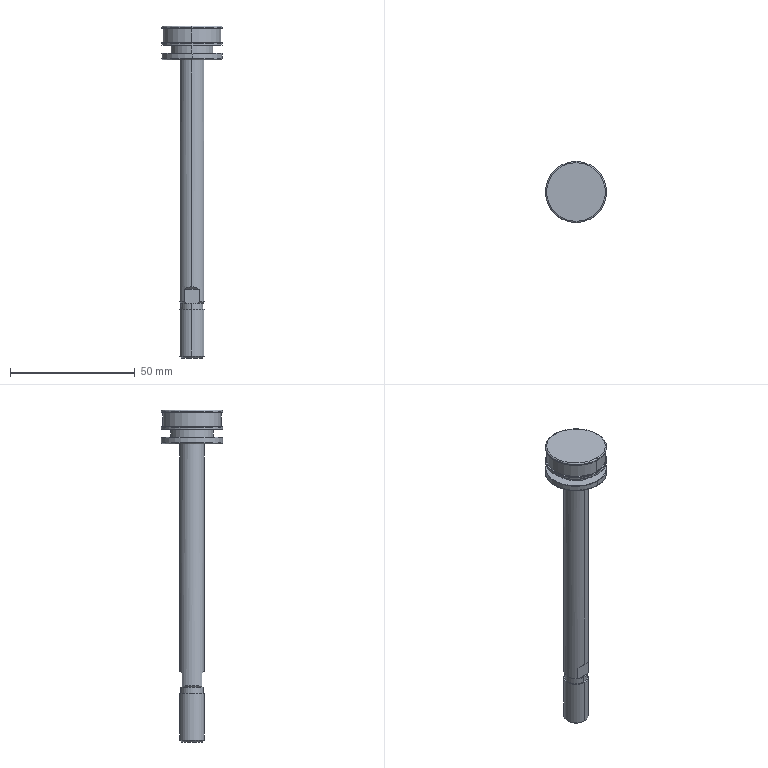Component | SolidWorks | MF_25x50_S_U_M_2_0-1_MF_25x50_S_U_r-1 | 1 solid | 50 faces | box 24.5 x 24.5 x 133 mm | volume 14640 mm3 | cylinder 16 | plane 14 | cone 12 | torus 8 | commonest cylinder face diameters 24.5 x6 10 x4 23.3 x2 17 x2 9 x2
build123d program:
from build123d import *

# Parameters (mm, degrees)
CUT_EXTRUDE1_DEPTH      = 5
CUT_EXTRUDE1_DEPTH_BACK = 5


with BuildPart() as part:
    # Sketch1 → Revolve1 (revolve)
    with BuildSketch(Plane.XY, mode=Mode.PRIVATE) as revolve1_sk:
        with BuildLine():
            Line((-45, 0), (-45, 4.233))
            Line((-45, 4.233), (-44.233, 5))
            Line((-44.233, 5), (-25.5, 5))
            Line((-25.5, 5), (-25.5, 4.5))
            Line((-25.5, 4.5), (-23, 4.5))
            Line((-23, 4.5), (-22.5, 5))
            Line((-22.5, 5), (74.4, 5))
            Line((74.4, 5), (74.4, 11.75))
            ThreePointArc((74.4, 11.75), (74.546, 12.104), (74.9, 12.25))
            Line((74.9, 12.25), (76.9, 12.25))
            Line((76.9, 12.25), (77, 12.15))
            Line((77, 12.15), (77, 8.5))
            Line((77, 8.5), (80.2, 8.5))
            Line((80.2, 8.5), (80.2, 12.15))
            Line((80.2, 12.15), (80.3, 12.25))
            Line((80.3, 12.25), (81.1, 12.25))
            Line((81.1, 12.25), (81.2, 12.15))
            Line((81.2, 12.15), (81.2, 11.75))
            ThreePointArc((81.2, 11.75), (81.229, 11.679), (81.3, 11.65))
            Line((81.3, 11.65), (86.9, 11.65))
            ThreePointArc((86.9, 11.65), (86.971, 11.679), (87, 11.75))
            Line((87, 11.75), (87, 12.15))
            Line((87, 12.15), (87.1, 12.25))
            Line((87.1, 12.25), (87.5, 12.25))
            ThreePointArc((87.5, 12.25), (87.854, 12.104), (88, 11.75))
            Line((88, 11.75), (88, 0))
            Line((88, 0), (-45, 0))
        make_face()
    revolve(revolve1_sk.sketch.rotate(Axis((88, 0, 0), (-1, 0, 0)), 270), axis=Axis((88, 0, 0), (-1, 0, 0)))

    # Sketch2 → Cut-Extrude1 (cut, two sides: drawn at the far end of the back side and taken through both)
    with BuildSketch(Plane(origin=(0, 0, 0), x_dir=(1, 0, 0), z_dir=(0, 1, 0)).offset(-CUT_EXTRUDE1_DEPTH_BACK)):
        Polygon((-55, 15), (-55, -15), (-6.5, -15), (-17.5, -4), (-23, -4), (-23, -5), (-45, -5), (-45, 5), (-23, 5), (-23, 4), (-17.5, 4), (-6.5, 15), align=None)
    extrude(amount=CUT_EXTRUDE1_DEPTH + CUT_EXTRUDE1_DEPTH_BACK, mode=Mode.SUBTRACT)


solid = part.part

# Placed as in the assembly
solid = solid.moved(Location((-102.5, -29.5, 213), (90, 0, 90)))